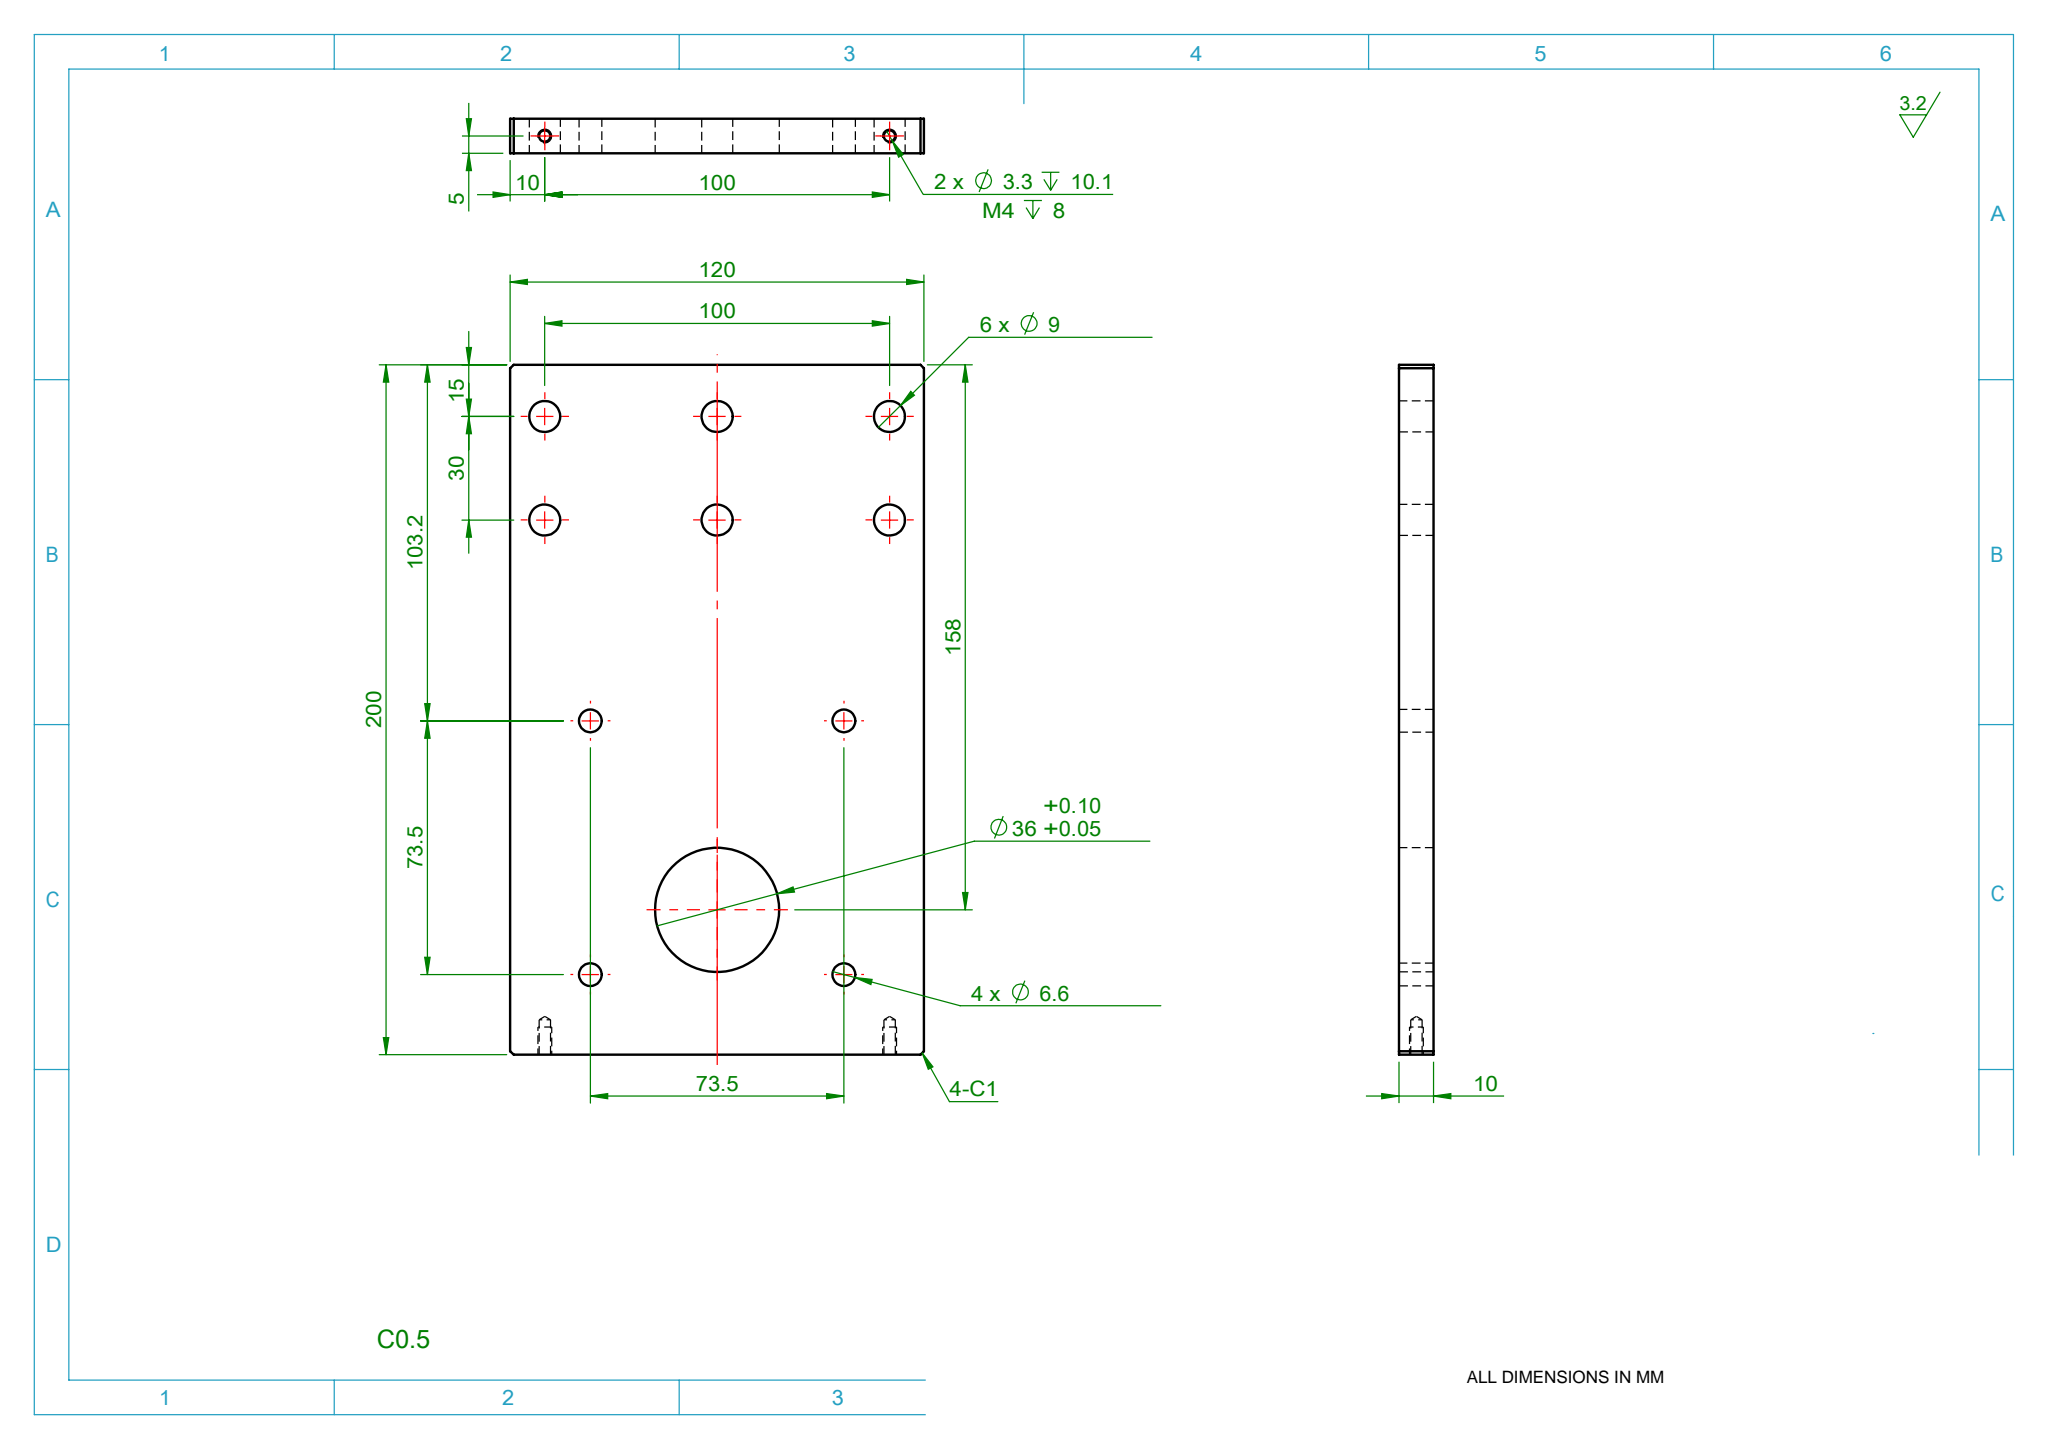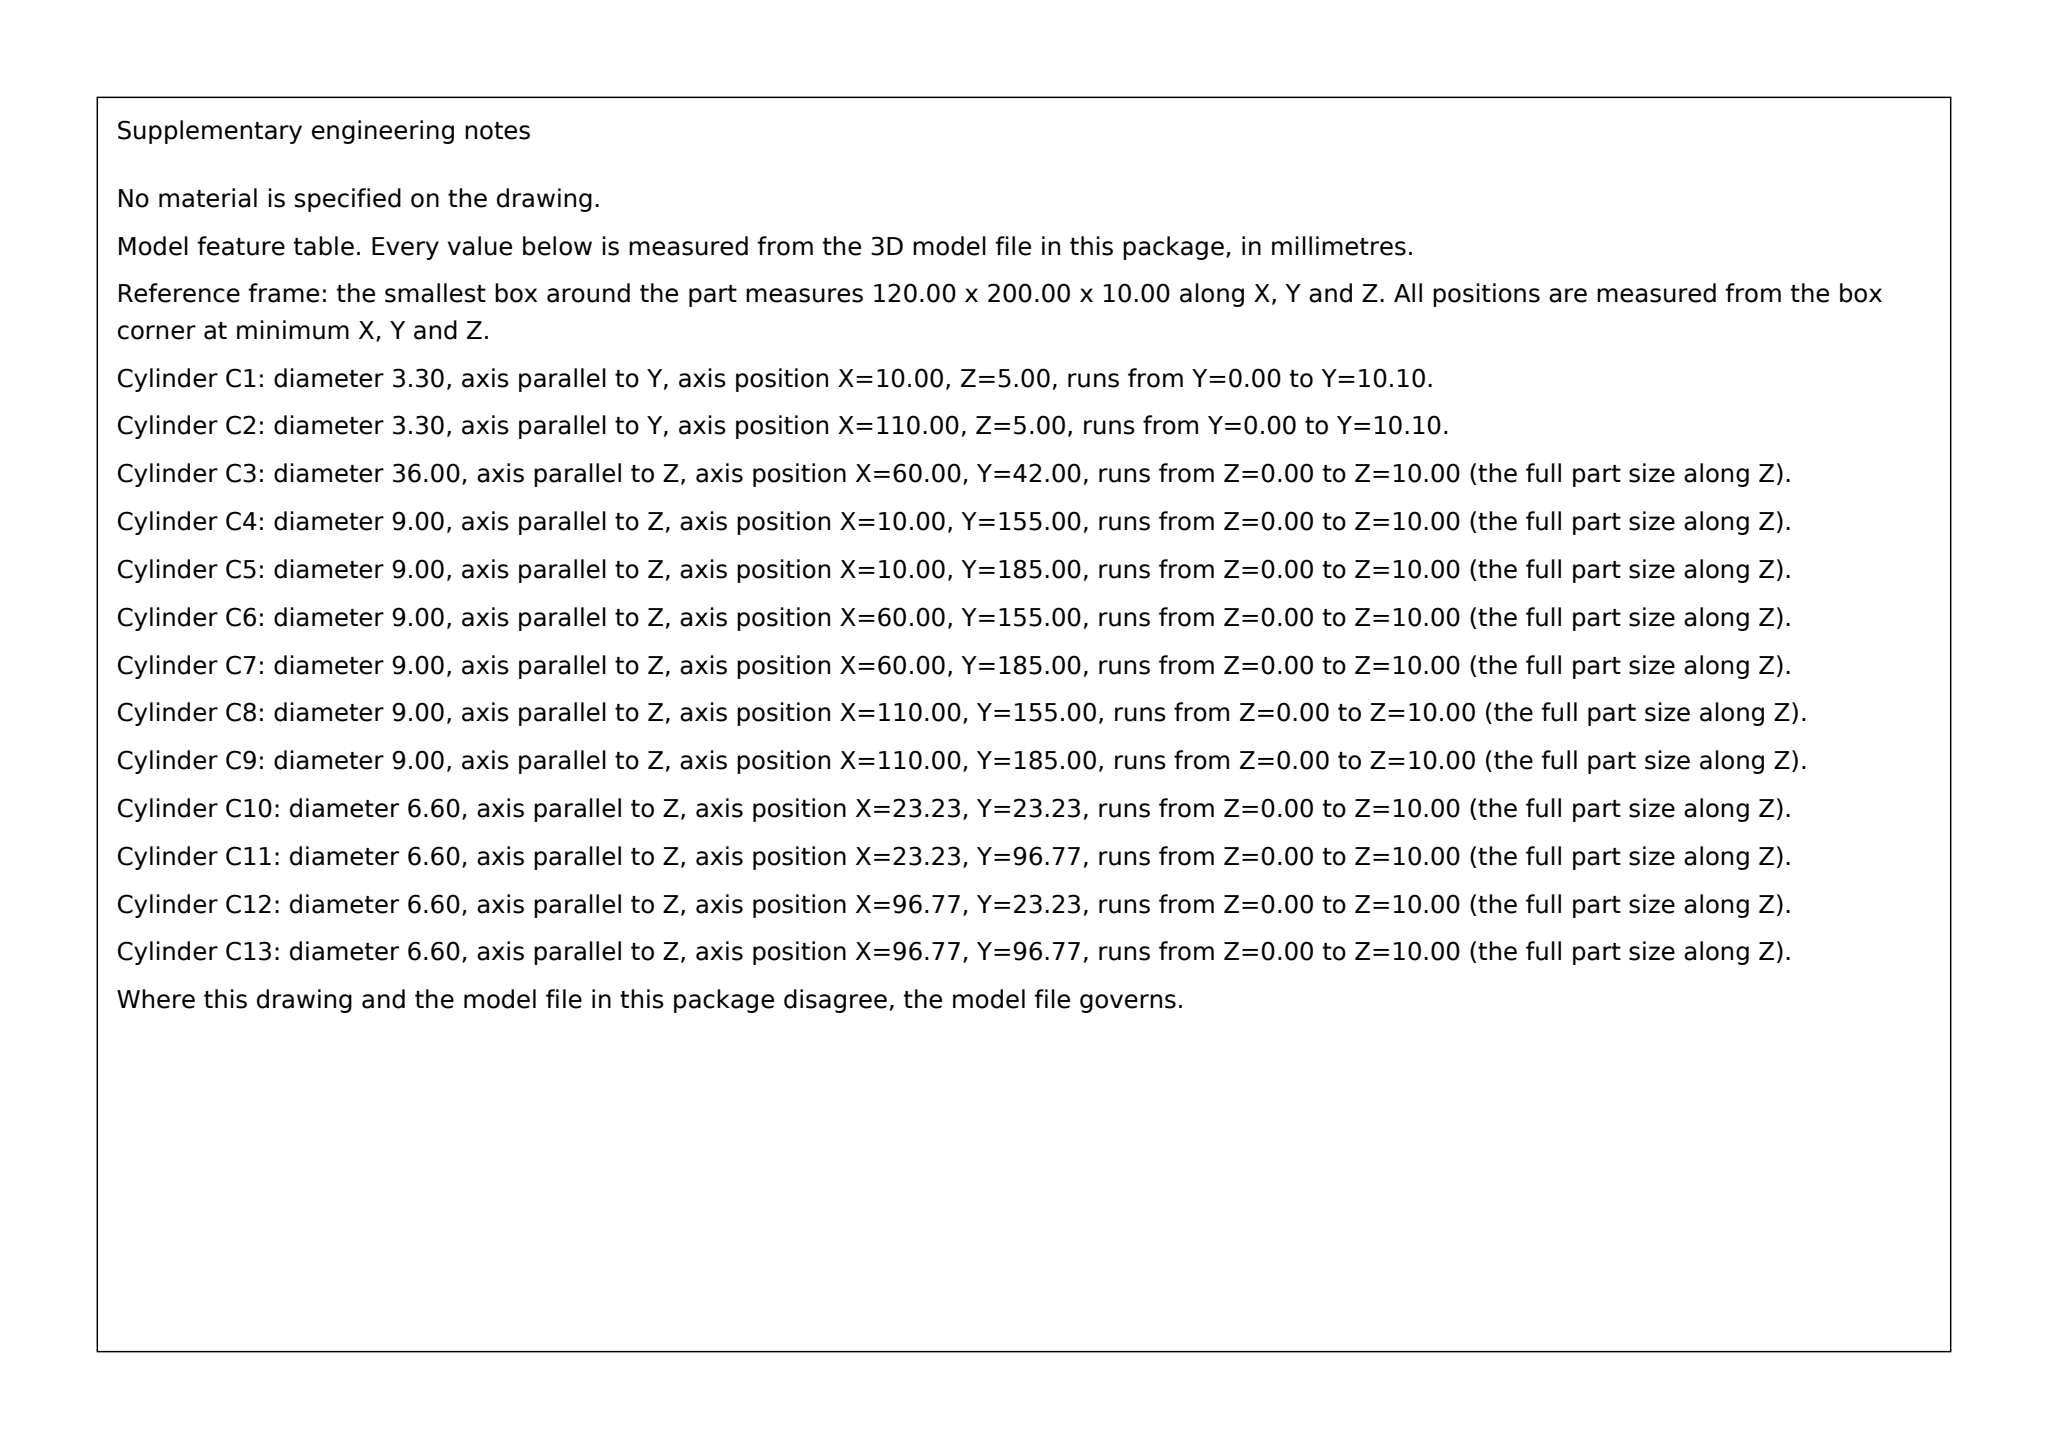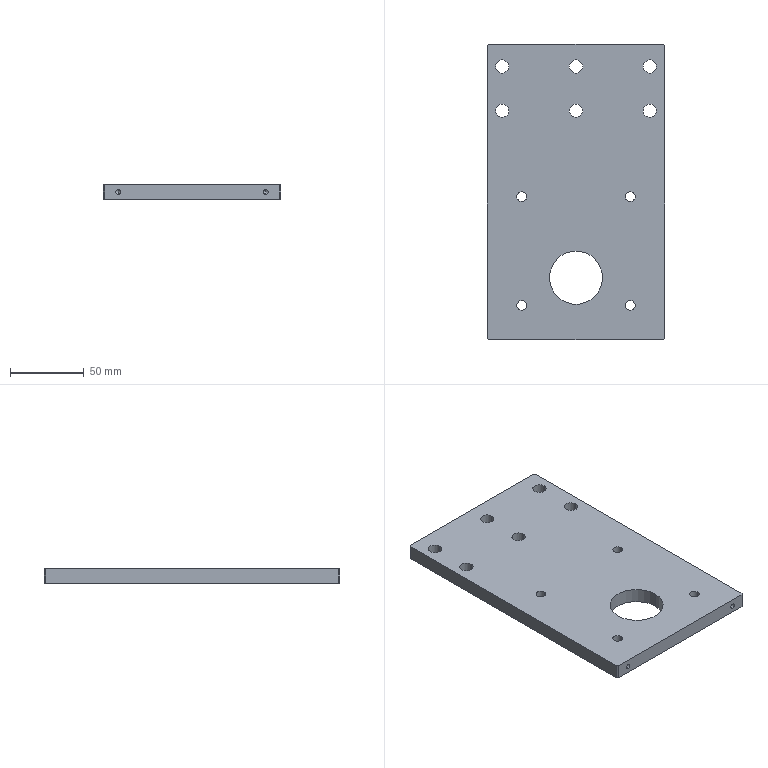Part | SolidWorks | mm | 1 solid | 40 faces | box 120 x 200 x 10 mm | volume 224437 mm3 | cylinder 26 | plane 10 | cone 4 | commonest cylinder face diameters 9 x12 6.6 x8 3.3 x4 36 x2
build123d program:
from build123d import *

# Parameters (mm, degrees)
SKETCH1_W             = 120
SKETCH1_H             = 200
BOSS_EXTRUDE1_DEPTH   = 10
M8_CLEARANCE_HOLE1_D  = 9
CHAMFER1_SIZE         = 1
M6_CLEARANCE_HOLE1_D  = 6.6
SKETCH6_R             = 18
CUT_EXTRUDE1_DEPTH    = 118.047
M4_TAPPED_HOLE1_D     = 3.3
M4_TAPPED_HOLE1_DEPTH = 10.1
M4_TAPPED_HOLE1_TIP   = 0.9914


with BuildPart() as part:
    # Sketch1 → Boss-Extrude1 (new body)
    with BuildSketch(Plane.XY):
        Rectangle(SKETCH1_W, SKETCH1_H)
    extrude(amount=BOSS_EXTRUDE1_DEPTH)

    # M8 Clearance Hole1 (through all)
    with Locations(Plane.XY.offset(10)):
        with Locations((-50, 85), (0, 85), (50, 85), (-50, 55), (0, 55), (50, 55)):
            Hole(M8_CLEARANCE_HOLE1_D / 2)

    # Chamfer1
    chamfer1_edges = [part.edges().sort_by_distance(p)[0] for p in [
        (60, -100, 5),
        (-60, -100, 5),
        (-60, 100, 5),
        (60, 100, 5),
    ]]
    chamfer(chamfer1_edges, length=CHAMFER1_SIZE)

    # M6 Clearance Hole1 (through all)
    with Locations(Plane.XY.offset(10)):
        with Locations((-36.77, -3.23), (36.77, -3.23), (-36.77, -76.77), (36.77, -76.77)):
            Hole(M6_CLEARANCE_HOLE1_D / 2)

    # Sketch6 → Cut-Extrude1 (cut, through all)
    with BuildSketch(Plane.XY.offset(10)):
        with Locations((0, -58)):
            Circle(SKETCH6_R)
    extrude(amount=-CUT_EXTRUDE1_DEPTH, mode=Mode.SUBTRACT)

    # M4 Tapped Hole1
    with Locations(Plane(origin=(0, -100, 0), x_dir=(-1, 0, 0), z_dir=(0, -1, 0))):
        with Locations((50, -5), (-50, -5)):
            Hole(M4_TAPPED_HOLE1_D / 2, depth=M4_TAPPED_HOLE1_DEPTH)
            with Locations((0, 0, -(M4_TAPPED_HOLE1_DEPTH + M4_TAPPED_HOLE1_TIP / 2))):  # 118° drill point
                Cone(0, M4_TAPPED_HOLE1_D / 2, M4_TAPPED_HOLE1_TIP, mode=Mode.SUBTRACT)


solid = part.part